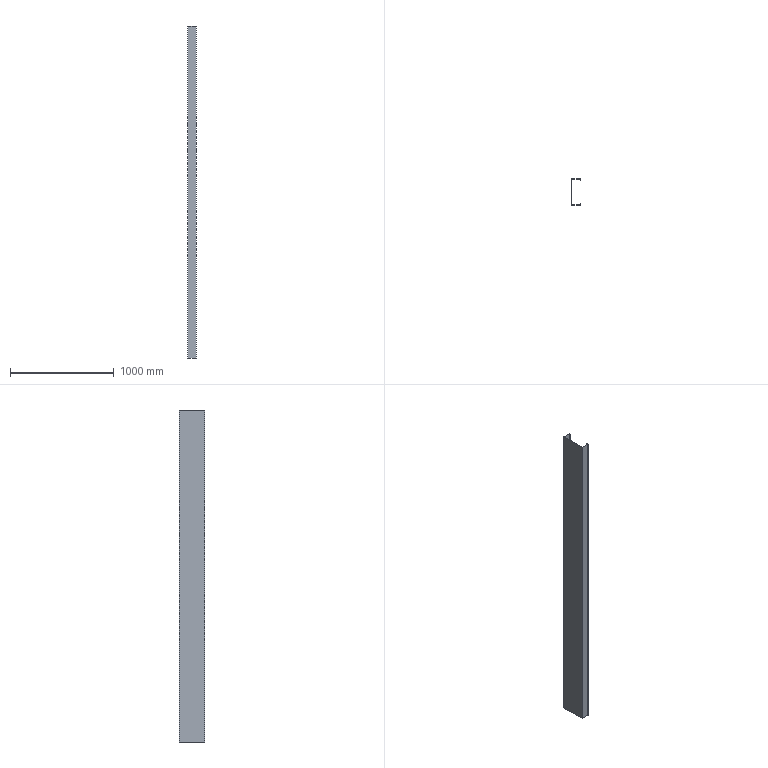Component | NX | DS4 | 1 solid | 14 faces | volume 2079945 mm3 | plane 14